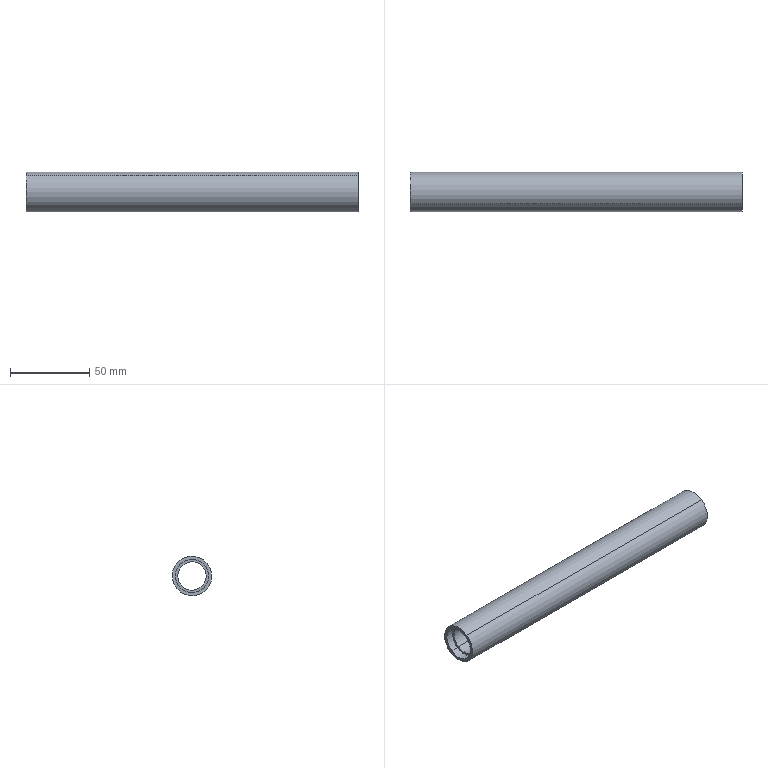Component | SolidWorks | GuideWheelAssembly3-1_Roller2-1 | 1 solid | 12 faces | box 210 x 25 x 25 mm | volume 48726 mm3 | cylinder 8 | plane 4 | commonest cylinder face diameters 21 x4 18 x2 25 x2
build123d program:
from build123d import *


with BuildPart() as part:
    # Sketch1 → Revolve1 (revolve)
    with BuildSketch(Plane.XY, mode=Mode.PRIVATE) as revolve1_sk:
        Polygon((0, 10.5), (5, 10.5), (5, 9), (205, 9), (205, 10.5), (210, 10.5), (210, 12.5), (0, 12.5), align=None)
    revolve(revolve1_sk.sketch.rotate(Axis((-1300.924, 0, 0), (1, 0, 0)), 90), axis=Axis((-1300.924, 0, 0), (1, 0, 0)))


solid = part.part

# Placed as in the assembly
solid = solid.moved(Location((-499.97, -235, 30), (0, 0, 0)))
STEP:
#1=CARTESIAN_POINT('',(-11.613,-9.011,0.8454));
#2=VERTEX_POINT('',#1);
#3=CARTESIAN_POINT('',(-11.613,-9.493,1.517));
#4=VERTEX_POINT('',#3);
#5=CARTESIAN_POINT('',(-11.613,-9.252,1.181));
#6=DIRECTION('',(1.,0.,0.));
#7=DIRECTION('',(0.,-0.5836,0.812));
#8=AXIS2_PLACEMENT_3D('',#5,#6,#7);
#9=CIRCLE('',#8,0.4134);
#10=EDGE_CURVE('',#2,#4,#9,.T.);
#11=ORIENTED_EDGE('',*,*,#10,.F.);
#12=CARTESIAN_POINT('',(-11.416,-9.011,0.8454));
#13=VERTEX_POINT('',#12);
#14=CARTESIAN_POINT('',(39.801,-9.011,0.8454));
#15=DIRECTION('',(1.,0.,0.));
#16=VECTOR('',#15,39.37);
#17=LINE('',#14,#16);
#18=EDGE_CURVE('',#2,#13,#17,.T.);
#19=ORIENTED_EDGE('',*,*,#18,.T.);
#20=CARTESIAN_POINT('',(-11.416,-9.493,1.517));
#21=VERTEX_POINT('',#20);
#22=CARTESIAN_POINT('',(-11.416,-9.252,1.181));
#23=DIRECTION('',(1.,0.,0.));
#24=DIRECTION('',(0.,-0.5836,0.812));
#25=AXIS2_PLACEMENT_3D('',#22,#23,#24);
#26=CIRCLE('',#25,0.4134);
#27=EDGE_CURVE('',#13,#21,#26,.T.);
#28=ORIENTED_EDGE('',*,*,#27,.T.);
#29=CARTESIAN_POINT('',(39.801,-9.493,1.517));
#30=DIRECTION('',(1.,0.,0.));
#31=VECTOR('',#30,39.37);
#32=LINE('',#29,#31);
#33=EDGE_CURVE('',#4,#21,#32,.T.);
#34=ORIENTED_EDGE('',*,*,#33,.F.);
#35=EDGE_LOOP('',(#11,#19,#28,#34));
#36=FACE_OUTER_BOUND('',#35,.T.);
#37=CARTESIAN_POINT('',(39.801,-9.252,1.181));
#38=DIRECTION('',(1.,0.,0.));
#39=DIRECTION('',(0.,-0.5836,0.812));
#40=AXIS2_PLACEMENT_3D('',#37,#38,#39);
#41=CYLINDRICAL_SURFACE('',#40,0.4134);
#42=ADVANCED_FACE('',(#36),#41,.F.);
#43=CARTESIAN_POINT('',(-19.487,-9.045,0.8934));
#44=VERTEX_POINT('',#43);
#45=CARTESIAN_POINT('',(-19.487,-9.459,1.469));
#46=VERTEX_POINT('',#45);
#47=CARTESIAN_POINT('',(-19.487,-9.252,1.181));
#48=DIRECTION('',(1.,0.,0.));
#49=DIRECTION('',(0.,-0.5836,0.812));
#50=AXIS2_PLACEMENT_3D('',#47,#48,#49);
#51=CIRCLE('',#50,0.3543);
#52=EDGE_CURVE('',#44,#46,#51,.T.);
#53=ORIENTED_EDGE('',*,*,#52,.F.);
#54=CARTESIAN_POINT('',(-11.613,-9.045,0.8934));
#55=VERTEX_POINT('',#54);
#56=CARTESIAN_POINT('',(39.801,-9.045,0.8934));
#57=DIRECTION('',(1.,0.,0.));
#58=VECTOR('',#57,39.37);
#59=LINE('',#56,#58);
#60=EDGE_CURVE('',#44,#55,#59,.T.);
#61=ORIENTED_EDGE('',*,*,#60,.T.);
#62=CARTESIAN_POINT('',(-11.613,-9.459,1.469));
#63=VERTEX_POINT('',#62);
#64=CARTESIAN_POINT('',(-11.613,-9.252,1.181));
#65=DIRECTION('',(1.,0.,0.));
#66=DIRECTION('',(0.,-0.5836,0.812));
#67=AXIS2_PLACEMENT_3D('',#64,#65,#66);
#68=CIRCLE('',#67,0.3543);
#69=EDGE_CURVE('',#55,#63,#68,.T.);
#70=ORIENTED_EDGE('',*,*,#69,.T.);
#71=CARTESIAN_POINT('',(39.801,-9.459,1.469));
#72=DIRECTION('',(1.,0.,0.));
#73=VECTOR('',#72,39.37);
#74=LINE('',#71,#73);
#75=EDGE_CURVE('',#46,#63,#74,.T.);
#76=ORIENTED_EDGE('',*,*,#75,.F.);
#77=EDGE_LOOP('',(#53,#61,#70,#76));
#78=FACE_OUTER_BOUND('',#77,.T.);
#79=CARTESIAN_POINT('',(39.801,-9.252,1.181));
#80=DIRECTION('',(1.,0.,0.));
#81=DIRECTION('',(0.,-0.5836,0.812));
#82=AXIS2_PLACEMENT_3D('',#79,#80,#81);
#83=CYLINDRICAL_SURFACE('',#82,0.3543);
#84=ADVANCED_FACE('',(#78),#83,.F.);
#85=CARTESIAN_POINT('',(-19.684,-9.011,0.8454));
#86=VERTEX_POINT('',#85);
#87=CARTESIAN_POINT('',(-19.684,-9.493,1.517));
#88=VERTEX_POINT('',#87);
#89=CARTESIAN_POINT('',(-19.684,-9.252,1.181));
#90=DIRECTION('',(1.,0.,0.));
#91=DIRECTION('',(0.,-0.5836,0.812));
#92=AXIS2_PLACEMENT_3D('',#89,#90,#91);
#93=CIRCLE('',#92,0.4134);
#94=EDGE_CURVE('',#86,#88,#93,.T.);
#95=ORIENTED_EDGE('',*,*,#94,.F.);
#96=CARTESIAN_POINT('',(-19.487,-9.011,0.8454));
#97=VERTEX_POINT('',#96);
#98=CARTESIAN_POINT('',(39.801,-9.011,0.8454));
#99=DIRECTION('',(1.,0.,0.));
#100=VECTOR('',#99,39.37);
#101=LINE('',#98,#100);
#102=EDGE_CURVE('',#86,#97,#101,.T.);
#103=ORIENTED_EDGE('',*,*,#102,.T.);
#104=CARTESIAN_POINT('',(-19.487,-9.493,1.517));
#105=VERTEX_POINT('',#104);
#106=CARTESIAN_POINT('',(-19.487,-9.252,1.181));
#107=DIRECTION('',(1.,0.,0.));
#108=DIRECTION('',(0.,-0.5836,0.812));
#109=AXIS2_PLACEMENT_3D('',#106,#107,#108);
#110=CIRCLE('',#109,0.4134);
#111=EDGE_CURVE('',#97,#105,#110,.T.);
#112=ORIENTED_EDGE('',*,*,#111,.T.);
#113=CARTESIAN_POINT('',(39.801,-9.493,1.517));
#114=DIRECTION('',(1.,0.,0.));
#115=VECTOR('',#114,39.37);
#116=LINE('',#113,#115);
#117=EDGE_CURVE('',#88,#105,#116,.T.);
#118=ORIENTED_EDGE('',*,*,#117,.F.);
#119=EDGE_LOOP('',(#95,#103,#112,#118));
#120=FACE_OUTER_BOUND('',#119,.T.);
#121=CARTESIAN_POINT('',(39.801,-9.252,1.181));
#122=DIRECTION('',(1.,0.,0.));
#123=DIRECTION('',(0.,-0.5836,0.812));
#124=AXIS2_PLACEMENT_3D('',#121,#122,#123);
#125=CYLINDRICAL_SURFACE('',#124,0.4134);
#126=ADVANCED_FACE('',(#120),#125,.F.);
#127=CARTESIAN_POINT('',(-19.684,-9.539,1.581));
#128=VERTEX_POINT('',#127);
#129=CARTESIAN_POINT('',(-19.684,-8.965,0.7815));
#130=VERTEX_POINT('',#129);
#131=CARTESIAN_POINT('',(-19.684,-9.252,1.181));
#132=DIRECTION('',(1.,0.,0.));
#133=DIRECTION('',(0.,-0.5836,0.812));
#134=AXIS2_PLACEMENT_3D('',#131,#132,#133);
#135=CIRCLE('',#134,0.4921);
#136=EDGE_CURVE('',#128,#130,#135,.T.);
#137=ORIENTED_EDGE('',*,*,#136,.T.);
#138=CARTESIAN_POINT('',(-11.416,-8.965,0.7815));
#139=VERTEX_POINT('',#138);
#140=CARTESIAN_POINT('',(39.801,-8.965,0.7815));
#141=DIRECTION('',(1.,0.,0.));
#142=VECTOR('',#141,39.37);
#143=LINE('',#140,#142);
#144=EDGE_CURVE('',#130,#139,#143,.T.);
#145=ORIENTED_EDGE('',*,*,#144,.T.);
#146=CARTESIAN_POINT('',(-11.416,-9.539,1.581));
#147=VERTEX_POINT('',#146);
#148=CARTESIAN_POINT('',(-11.416,-9.252,1.181));
#149=DIRECTION('',(1.,0.,0.));
#150=DIRECTION('',(0.,-0.5836,0.812));
#151=AXIS2_PLACEMENT_3D('',#148,#149,#150);
#152=CIRCLE('',#151,0.4921);
#153=EDGE_CURVE('',#147,#139,#152,.T.);
#154=ORIENTED_EDGE('',*,*,#153,.F.);
#155=CARTESIAN_POINT('',(39.801,-9.539,1.581));
#156=DIRECTION('',(1.,0.,0.));
#157=VECTOR('',#156,39.37);
#158=LINE('',#155,#157);
#159=EDGE_CURVE('',#128,#147,#158,.T.);
#160=ORIENTED_EDGE('',*,*,#159,.F.);
#161=EDGE_LOOP('',(#137,#145,#154,#160));
#162=FACE_OUTER_BOUND('',#161,.T.);
#163=CARTESIAN_POINT('',(39.801,-9.252,1.181));
#164=DIRECTION('',(1.,0.,0.));
#165=DIRECTION('',(0.,-0.5836,0.812));
#166=AXIS2_PLACEMENT_3D('',#163,#164,#165);
#167=CYLINDRICAL_SURFACE('',#166,0.4921);
#168=ADVANCED_FACE('',(#162),#167,.T.);
#169=CARTESIAN_POINT('',(-11.416,-9.252,1.181));
#170=DIRECTION('',(1.,0.,0.));
#171=DIRECTION('',(0.,-0.5836,0.812));
#172=AXIS2_PLACEMENT_3D('',#169,#170,#171);
#173=CIRCLE('',#172,0.4134);
#174=EDGE_CURVE('',#21,#13,#173,.T.);
#175=ORIENTED_EDGE('',*,*,#174,.F.);
#176=ORIENTED_EDGE('',*,*,#27,.F.);
#177=EDGE_LOOP('',(#175,#176));
#178=FACE_BOUND('',#177,.T.);
#179=ORIENTED_EDGE('',*,*,#153,.T.);
#180=CARTESIAN_POINT('',(-11.416,-9.252,1.181));
#181=DIRECTION('',(1.,0.,0.));
#182=DIRECTION('',(0.,-0.5836,0.812));
#183=AXIS2_PLACEMENT_3D('',#180,#181,#182);
#184=CIRCLE('',#183,0.4921);
#185=EDGE_CURVE('',#139,#147,#184,.T.);
#186=ORIENTED_EDGE('',*,*,#185,.T.);
#187=EDGE_LOOP('',(#179,#186));
#188=FACE_OUTER_BOUND('',#187,.T.);
#189=CARTESIAN_POINT('',(-11.416,-9.588,0.9398));
#190=DIRECTION('',(-1.,-0.,-0.));
#191=DIRECTION('',(-0.,0.5836,-0.812));
#192=AXIS2_PLACEMENT_3D('',#189,#190,#191);
#193=PLANE('',#192);
#194=ADVANCED_FACE('',(#178,#188),#193,.F.);
#195=ORIENTED_EDGE('',*,*,#144,.F.);
#196=CARTESIAN_POINT('',(-19.684,-9.252,1.181));
#197=DIRECTION('',(1.,0.,0.));
#198=DIRECTION('',(0.,-0.5836,0.812));
#199=AXIS2_PLACEMENT_3D('',#196,#197,#198);
#200=CIRCLE('',#199,0.4921);
#201=EDGE_CURVE('',#130,#128,#200,.T.);
#202=ORIENTED_EDGE('',*,*,#201,.T.);
#203=ORIENTED_EDGE('',*,*,#159,.T.);
#204=ORIENTED_EDGE('',*,*,#185,.F.);
#205=EDGE_LOOP('',(#195,#202,#203,#204));
#206=FACE_OUTER_BOUND('',#205,.T.);
#207=CARTESIAN_POINT('',(39.801,-9.252,1.181));
#208=DIRECTION('',(1.,0.,0.));
#209=DIRECTION('',(0.,-0.5836,0.812));
#210=AXIS2_PLACEMENT_3D('',#207,#208,#209);
#211=CYLINDRICAL_SURFACE('',#210,0.4921);
#212=ADVANCED_FACE('',(#206),#211,.T.);
#213=ORIENTED_EDGE('',*,*,#136,.F.);
#214=ORIENTED_EDGE('',*,*,#201,.F.);
#215=EDGE_LOOP('',(#213,#214));
#216=FACE_OUTER_BOUND('',#215,.T.);
#217=CARTESIAN_POINT('',(-19.684,-9.252,1.181));
#218=DIRECTION('',(1.,0.,0.));
#219=DIRECTION('',(0.,-0.5836,0.812));
#220=AXIS2_PLACEMENT_3D('',#217,#218,#219);
#221=CIRCLE('',#220,0.4134);
#222=EDGE_CURVE('',#88,#86,#221,.T.);
#223=ORIENTED_EDGE('',*,*,#222,.T.);
#224=ORIENTED_EDGE('',*,*,#94,.T.);
#225=EDGE_LOOP('',(#223,#224));
#226=FACE_BOUND('',#225,.T.);
#227=CARTESIAN_POINT('',(-19.684,-9.652,0.8939));
#228=DIRECTION('',(1.,0.,0.));
#229=DIRECTION('',(0.,-0.5836,0.812));
#230=AXIS2_PLACEMENT_3D('',#227,#228,#229);
#231=PLANE('',#230);
#232=ADVANCED_FACE('',(#216,#226),#231,.F.);
#233=ORIENTED_EDGE('',*,*,#102,.F.);
#234=ORIENTED_EDGE('',*,*,#222,.F.);
#235=ORIENTED_EDGE('',*,*,#117,.T.);
#236=CARTESIAN_POINT('',(-19.487,-9.252,1.181));
#237=DIRECTION('',(1.,0.,0.));
#238=DIRECTION('',(0.,-0.5836,0.812));
#239=AXIS2_PLACEMENT_3D('',#236,#237,#238);
#240=CIRCLE('',#239,0.4134);
#241=EDGE_CURVE('',#105,#97,#240,.T.);
#242=ORIENTED_EDGE('',*,*,#241,.T.);
#243=EDGE_LOOP('',(#233,#234,#235,#242));
#244=FACE_OUTER_BOUND('',#243,.T.);
#245=CARTESIAN_POINT('',(39.801,-9.252,1.181));
#246=DIRECTION('',(1.,0.,0.));
#247=DIRECTION('',(0.,-0.5836,0.812));
#248=AXIS2_PLACEMENT_3D('',#245,#246,#247);
#249=CYLINDRICAL_SURFACE('',#248,0.4134);
#250=ADVANCED_FACE('',(#244),#249,.F.);
#251=ORIENTED_EDGE('',*,*,#241,.F.);
#252=ORIENTED_EDGE('',*,*,#111,.F.);
#253=EDGE_LOOP('',(#251,#252));
#254=FACE_OUTER_BOUND('',#253,.T.);
#255=CARTESIAN_POINT('',(-19.487,-9.252,1.181));
#256=DIRECTION('',(1.,0.,0.));
#257=DIRECTION('',(0.,-0.5836,0.812));
#258=AXIS2_PLACEMENT_3D('',#255,#256,#257);
#259=CIRCLE('',#258,0.3543);
#260=EDGE_CURVE('',#46,#44,#259,.T.);
#261=ORIENTED_EDGE('',*,*,#260,.T.);
#262=ORIENTED_EDGE('',*,*,#52,.T.);
#263=EDGE_LOOP('',(#261,#262));
#264=FACE_BOUND('',#263,.T.);
#265=CARTESIAN_POINT('',(-19.487,-9.54,0.9743));
#266=DIRECTION('',(1.,0.,0.));
#267=DIRECTION('',(0.,-0.5836,0.812));
#268=AXIS2_PLACEMENT_3D('',#265,#266,#267);
#269=PLANE('',#268);
#270=ADVANCED_FACE('',(#254,#264),#269,.F.);
#271=ORIENTED_EDGE('',*,*,#60,.F.);
#272=ORIENTED_EDGE('',*,*,#260,.F.);
#273=ORIENTED_EDGE('',*,*,#75,.T.);
#274=CARTESIAN_POINT('',(-11.613,-9.252,1.181));
#275=DIRECTION('',(1.,0.,0.));
#276=DIRECTION('',(0.,-0.5836,0.812));
#277=AXIS2_PLACEMENT_3D('',#274,#275,#276);
#278=CIRCLE('',#277,0.3543);
#279=EDGE_CURVE('',#63,#55,#278,.T.);
#280=ORIENTED_EDGE('',*,*,#279,.T.);
#281=EDGE_LOOP('',(#271,#272,#273,#280));
#282=FACE_OUTER_BOUND('',#281,.T.);
#283=CARTESIAN_POINT('',(39.801,-9.252,1.181));
#284=DIRECTION('',(1.,0.,0.));
#285=DIRECTION('',(0.,-0.5836,0.812));
#286=AXIS2_PLACEMENT_3D('',#283,#284,#285);
#287=CYLINDRICAL_SURFACE('',#286,0.3543);
#288=ADVANCED_FACE('',(#282),#287,.F.);
#289=ORIENTED_EDGE('',*,*,#279,.F.);
#290=ORIENTED_EDGE('',*,*,#69,.F.);
#291=EDGE_LOOP('',(#289,#290));
#292=FACE_BOUND('',#291,.T.);
#293=CARTESIAN_POINT('',(-11.613,-9.252,1.181));
#294=DIRECTION('',(1.,0.,0.));
#295=DIRECTION('',(0.,-0.5836,0.812));
#296=AXIS2_PLACEMENT_3D('',#293,#294,#295);
#297=CIRCLE('',#296,0.4134);
#298=EDGE_CURVE('',#4,#2,#297,.T.);
#299=ORIENTED_EDGE('',*,*,#298,.T.);
#300=ORIENTED_EDGE('',*,*,#10,.T.);
#301=EDGE_LOOP('',(#299,#300));
#302=FACE_OUTER_BOUND('',#301,.T.);
#303=CARTESIAN_POINT('',(-11.613,-9.588,0.9398));
#304=DIRECTION('',(-1.,-0.,-0.));
#305=DIRECTION('',(-0.,0.5836,-0.812));
#306=AXIS2_PLACEMENT_3D('',#303,#304,#305);
#307=PLANE('',#306);
#308=ADVANCED_FACE('',(#292,#302),#307,.F.);
#309=ORIENTED_EDGE('',*,*,#18,.F.);
#310=ORIENTED_EDGE('',*,*,#298,.F.);
#311=ORIENTED_EDGE('',*,*,#33,.T.);
#312=ORIENTED_EDGE('',*,*,#174,.T.);
#313=EDGE_LOOP('',(#309,#310,#311,#312));
#314=FACE_OUTER_BOUND('',#313,.T.);
#315=CARTESIAN_POINT('',(39.801,-9.252,1.181));
#316=DIRECTION('',(1.,0.,0.));
#317=DIRECTION('',(0.,-0.5836,0.812));
#318=AXIS2_PLACEMENT_3D('',#315,#316,#317);
#319=CYLINDRICAL_SURFACE('',#318,0.4134);
#320=ADVANCED_FACE('',(#314),#319,.F.);
#321=CLOSED_SHELL('',(#42,#84,#126,#168,#194,#212,#232,#250,#270,#288,#308,#320));
#322=MANIFOLD_SOLID_BREP('',#321);
#323=CARTESIAN_POINT('',(0.,0.,0.));
#324=DIRECTION('',(0.,0.,1.));
#325=DIRECTION('',(1.,0.,0.));
#326=AXIS2_PLACEMENT_3D('',#323,#324,#325);
#327=(LENGTH_UNIT()NAMED_UNIT(*)SI_UNIT($,.METRE.));
#328=LENGTH_MEASURE_WITH_UNIT(LENGTH_MEASURE(0.0254),#327);
#329=DIMENSIONAL_EXPONENTS(1.,0.,0.,0.,0.,0.,0.);
#330=(CONVERSION_BASED_UNIT('',#328)LENGTH_UNIT()NAMED_UNIT(#329));
#331=UNCERTAINTY_MEASURE_WITH_UNIT(LENGTH_MEASURE(0.00001),#330,'','');
#332=(NAMED_UNIT(*)PLANE_ANGLE_UNIT()SI_UNIT($,.RADIAN.));
#333=(NAMED_UNIT(*)SI_UNIT($,.STERADIAN.)SOLID_ANGLE_UNIT());
#334=(GEOMETRIC_REPRESENTATION_CONTEXT(3)GLOBAL_UNCERTAINTY_ASSIGNED_CONTEXT((#331))GLOBAL_UNIT_ASSIGNED_CONTEXT((#330,#332,#333))REPRESENTATION_CONTEXT('',''));
#335=ADVANCED_BREP_SHAPE_REPRESENTATION('',(#322,#326),#334);
#336=COLOUR_RGB('',0.7922,0.8196,0.9333);
#337=FILL_AREA_STYLE_COLOUR('',#336);
#338=FILL_AREA_STYLE('',(#337));
#339=SURFACE_STYLE_FILL_AREA(#338);
#340=SURFACE_SIDE_STYLE('',(#339));
#341=SURFACE_STYLE_USAGE(.BOTH.,#340);
#342=PRESENTATION_STYLE_ASSIGNMENT((#341));
#343=STYLED_ITEM('',(#342),#322);
#344=(LENGTH_UNIT()NAMED_UNIT(*)SI_UNIT($,.METRE.));
#345=LENGTH_MEASURE_WITH_UNIT(LENGTH_MEASURE(0.0254),#344);
#346=DIMENSIONAL_EXPONENTS(1.,0.,0.,0.,0.,0.,0.);
#347=(CONVERSION_BASED_UNIT('',#345)LENGTH_UNIT()NAMED_UNIT(#346));
#348=UNCERTAINTY_MEASURE_WITH_UNIT(LENGTH_MEASURE(0.00001),#347,'','');
#349=(NAMED_UNIT(*)PLANE_ANGLE_UNIT()SI_UNIT($,.RADIAN.));
#350=(NAMED_UNIT(*)SI_UNIT($,.STERADIAN.)SOLID_ANGLE_UNIT());
#351=(GEOMETRIC_REPRESENTATION_CONTEXT(3)GLOBAL_UNCERTAINTY_ASSIGNED_CONTEXT((#348))GLOBAL_UNIT_ASSIGNED_CONTEXT((#347,#349,#350))REPRESENTATION_CONTEXT('',''));
#352=MECHANICAL_DESIGN_GEOMETRIC_PRESENTATION_REPRESENTATION('',(#343),#351);
#353=PRESENTATION_LAYER_ASSIGNMENT('','',(#343));